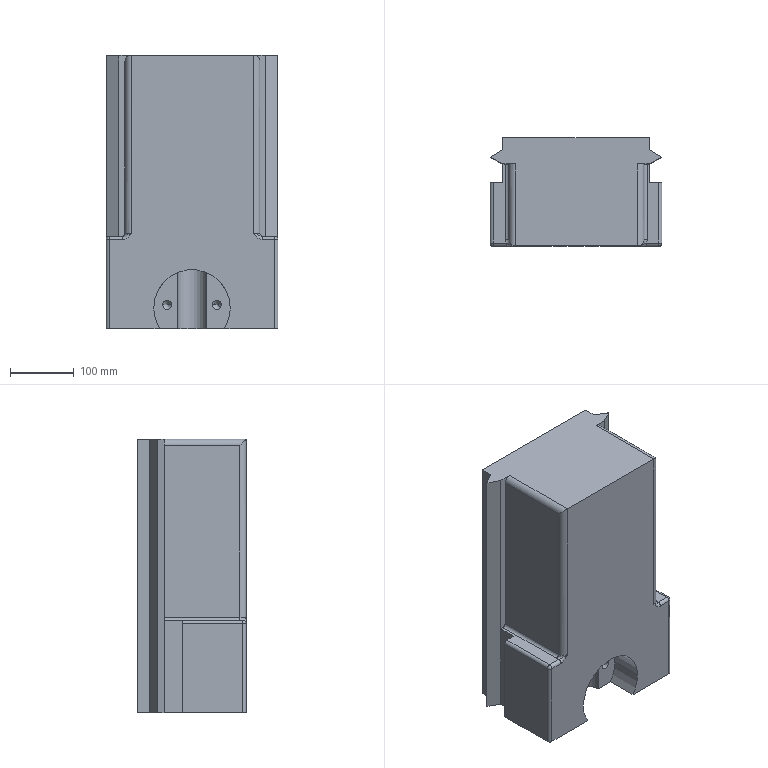Component | SolidWorks | Slider-1 | 1 solid | 57 faces | volume 16311184 mm3 | plane 25 | cylinder 22 | cone 4 | spline 4 | torus 1 | sphere 1 | commonest cylinder face diameters 10 x8 20 x5 14 x4 120 x3 45 x2